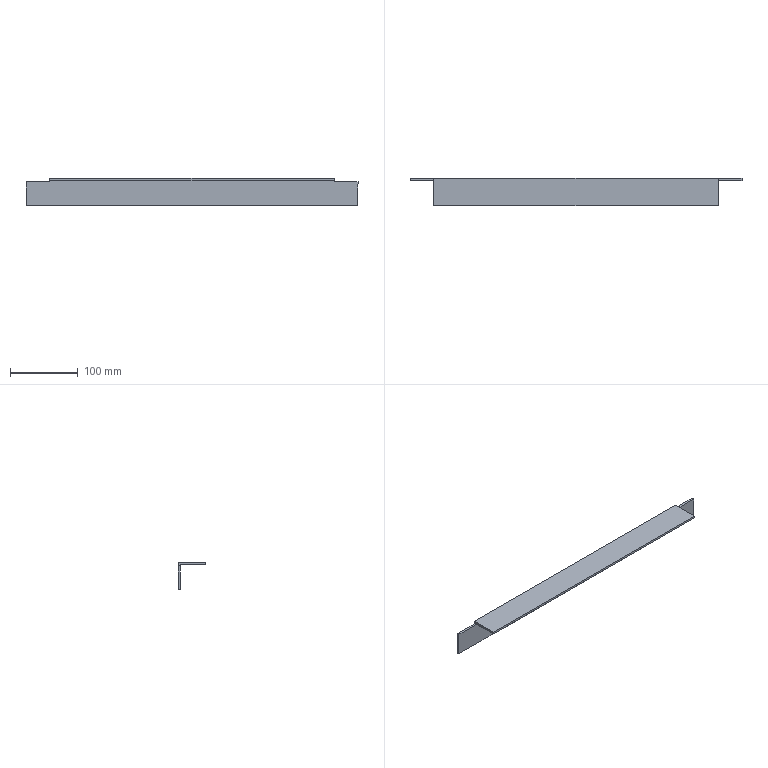Component | SolidWorks | LX-TSJ-13-1 | 1 solid | 12 faces | box 490 x 40 x 40 mm | volume 104370 mm3 | plane 12
STEP:
#1=COLOUR_RGB('',0.7922,0.8196,0.9333);
#2=FILL_AREA_STYLE_COLOUR('',#1);
#3=FILL_AREA_STYLE('',(#2));
#4=SURFACE_STYLE_FILL_AREA(#3);
#5=SURFACE_SIDE_STYLE('',(#4));
#6=SURFACE_STYLE_USAGE(.BOTH.,#5);
#7=PRESENTATION_STYLE_ASSIGNMENT((#6));
#8=CARTESIAN_POINT('',(2.637,-23.56,-6.468));
#9=VERTEX_POINT('',#8);
#10=CARTESIAN_POINT('',(-13.899,-23.56,-6.468));
#11=VERTEX_POINT('',#10);
#12=CARTESIAN_POINT('',(-15.276,-23.56,-6.468));
#13=DIRECTION('',(-1.,0.,0.));
#14=VECTOR('',#13,39.37);
#15=LINE('',#12,#14);
#16=EDGE_CURVE('',#9,#11,#15,.T.);
#17=ORIENTED_EDGE('',*,*,#16,.F.);
#18=CARTESIAN_POINT('',(2.637,-23.56,-6.665));
#19=VERTEX_POINT('',#18);
#20=CARTESIAN_POINT('',(2.637,-23.56,-8.043));
#21=DIRECTION('',(0.,0.,1.));
#22=VECTOR('',#21,39.37);
#23=LINE('',#20,#22);
#24=EDGE_CURVE('',#19,#9,#23,.T.);
#25=ORIENTED_EDGE('',*,*,#24,.F.);
#26=CARTESIAN_POINT('',(4.015,-23.56,-6.665));
#27=VERTEX_POINT('',#26);
#28=CARTESIAN_POINT('',(-15.276,-23.56,-6.665));
#29=DIRECTION('',(-1.,0.,0.));
#30=VECTOR('',#29,39.37);
#31=LINE('',#28,#30);
#32=EDGE_CURVE('',#27,#19,#31,.T.);
#33=ORIENTED_EDGE('',*,*,#32,.F.);
#34=CARTESIAN_POINT('',(4.015,-23.56,-8.043));
#35=VERTEX_POINT('',#34);
#36=CARTESIAN_POINT('',(4.015,-23.56,-8.043));
#37=DIRECTION('',(0.,0.,1.));
#38=VECTOR('',#37,39.37);
#39=LINE('',#36,#38);
#40=EDGE_CURVE('',#35,#27,#39,.T.);
#41=ORIENTED_EDGE('',*,*,#40,.F.);
#42=CARTESIAN_POINT('',(-15.276,-23.56,-8.043));
#43=VERTEX_POINT('',#42);
#44=CARTESIAN_POINT('',(-15.276,-23.56,-8.043));
#45=DIRECTION('',(1.,0.,-0.));
#46=VECTOR('',#45,39.37);
#47=LINE('',#44,#46);
#48=EDGE_CURVE('',#43,#35,#47,.T.);
#49=ORIENTED_EDGE('',*,*,#48,.F.);
#50=CARTESIAN_POINT('',(-15.276,-23.56,-6.665));
#51=VERTEX_POINT('',#50);
#52=CARTESIAN_POINT('',(-15.276,-23.56,-8.043));
#53=DIRECTION('',(-0.,0.,-1.));
#54=VECTOR('',#53,39.37);
#55=LINE('',#52,#54);
#56=EDGE_CURVE('',#51,#43,#55,.T.);
#57=ORIENTED_EDGE('',*,*,#56,.F.);
#58=CARTESIAN_POINT('',(-13.899,-23.56,-6.665));
#59=VERTEX_POINT('',#58);
#60=CARTESIAN_POINT('',(-15.276,-23.56,-6.665));
#61=DIRECTION('',(-1.,0.,0.));
#62=VECTOR('',#61,39.37);
#63=LINE('',#60,#62);
#64=EDGE_CURVE('',#59,#51,#63,.T.);
#65=ORIENTED_EDGE('',*,*,#64,.F.);
#66=CARTESIAN_POINT('',(-13.899,-23.56,-8.043));
#67=DIRECTION('',(-0.,0.,-1.));
#68=VECTOR('',#67,39.37);
#69=LINE('',#66,#68);
#70=EDGE_CURVE('',#11,#59,#69,.T.);
#71=ORIENTED_EDGE('',*,*,#70,.F.);
#72=EDGE_LOOP('',(#17,#25,#33,#41,#49,#57,#65,#71));
#73=FACE_OUTER_BOUND('',#72,.T.);
#74=CARTESIAN_POINT('',(-15.276,-23.56,-8.043));
#75=DIRECTION('',(0.,-1.,0.));
#76=DIRECTION('',(1.,0.,-0.));
#77=AXIS2_PLACEMENT_3D('',#74,#75,#76);
#78=PLANE('',#77);
#79=ADVANCED_FACE('',(#73),#78,.F.);
#80=ORIENTED_EDGE('',*,*,#16,.T.);
#81=CARTESIAN_POINT('',(-13.899,-25.134,-6.468));
#82=VERTEX_POINT('',#81);
#83=CARTESIAN_POINT('',(-13.899,-23.56,-6.468));
#84=DIRECTION('',(0.,1.,0.));
#85=VECTOR('',#84,39.37);
#86=LINE('',#83,#85);
#87=EDGE_CURVE('',#82,#11,#86,.T.);
#88=ORIENTED_EDGE('',*,*,#87,.F.);
#89=CARTESIAN_POINT('',(2.637,-25.134,-6.468));
#90=VERTEX_POINT('',#89);
#91=CARTESIAN_POINT('',(-15.276,-25.134,-6.468));
#92=DIRECTION('',(-1.,0.,0.));
#93=VECTOR('',#92,39.37);
#94=LINE('',#91,#93);
#95=EDGE_CURVE('',#90,#82,#94,.T.);
#96=ORIENTED_EDGE('',*,*,#95,.F.);
#97=CARTESIAN_POINT('',(2.637,-23.56,-6.468));
#98=DIRECTION('',(0.,-1.,0.));
#99=VECTOR('',#98,39.37);
#100=LINE('',#97,#99);
#101=EDGE_CURVE('',#9,#90,#100,.T.);
#102=ORIENTED_EDGE('',*,*,#101,.F.);
#103=EDGE_LOOP('',(#80,#88,#96,#102));
#104=FACE_OUTER_BOUND('',#103,.T.);
#105=CARTESIAN_POINT('',(-15.276,-23.56,-6.468));
#106=DIRECTION('',(-0.,0.,-1.));
#107=DIRECTION('',(-1.,0.,0.));
#108=AXIS2_PLACEMENT_3D('',#105,#106,#107);
#109=PLANE('',#108);
#110=ADVANCED_FACE('',(#104),#109,.F.);
#111=ORIENTED_EDGE('',*,*,#101,.T.);
#112=CARTESIAN_POINT('',(2.637,-25.134,-6.587));
#113=VERTEX_POINT('',#112);
#114=CARTESIAN_POINT('',(2.637,-25.134,-6.665));
#115=DIRECTION('',(0.,0.,1.));
#116=VECTOR('',#115,39.37);
#117=LINE('',#114,#116);
#118=EDGE_CURVE('',#113,#90,#117,.T.);
#119=ORIENTED_EDGE('',*,*,#118,.F.);
#120=CARTESIAN_POINT('',(2.637,-23.678,-6.587));
#121=VERTEX_POINT('',#120);
#122=CARTESIAN_POINT('',(2.637,-25.134,-6.587));
#123=DIRECTION('',(0.,-1.,0.));
#124=VECTOR('',#123,39.37);
#125=LINE('',#122,#124);
#126=EDGE_CURVE('',#121,#113,#125,.T.);
#127=ORIENTED_EDGE('',*,*,#126,.F.);
#128=CARTESIAN_POINT('',(2.637,-23.678,-6.665));
#129=VERTEX_POINT('',#128);
#130=CARTESIAN_POINT('',(2.637,-23.678,-6.665));
#131=DIRECTION('',(0.,0.,1.));
#132=VECTOR('',#131,39.37);
#133=LINE('',#130,#132);
#134=EDGE_CURVE('',#129,#121,#133,.T.);
#135=ORIENTED_EDGE('',*,*,#134,.F.);
#136=CARTESIAN_POINT('',(2.637,-25.134,-6.665));
#137=DIRECTION('',(0.,-1.,0.));
#138=VECTOR('',#137,39.37);
#139=LINE('',#136,#138);
#140=EDGE_CURVE('',#19,#129,#139,.T.);
#141=ORIENTED_EDGE('',*,*,#140,.F.);
#142=ORIENTED_EDGE('',*,*,#24,.T.);
#143=EDGE_LOOP('',(#111,#119,#127,#135,#141,#142));
#144=FACE_OUTER_BOUND('',#143,.T.);
#145=CARTESIAN_POINT('',(2.637,-25.134,-6.665));
#146=DIRECTION('',(-1.,0.,0.));
#147=DIRECTION('',(0.,0.,1.));
#148=AXIS2_PLACEMENT_3D('',#145,#146,#147);
#149=PLANE('',#148);
#150=ADVANCED_FACE('',(#144),#149,.F.);
#151=ORIENTED_EDGE('',*,*,#32,.T.);
#152=ORIENTED_EDGE('',*,*,#140,.T.);
#153=CARTESIAN_POINT('',(4.015,-23.678,-6.665));
#154=VERTEX_POINT('',#153);
#155=CARTESIAN_POINT('',(4.015,-23.678,-6.665));
#156=DIRECTION('',(1.,0.,-0.));
#157=VECTOR('',#156,39.37);
#158=LINE('',#155,#157);
#159=EDGE_CURVE('',#129,#154,#158,.T.);
#160=ORIENTED_EDGE('',*,*,#159,.T.);
#161=CARTESIAN_POINT('',(4.015,-23.56,-6.665));
#162=DIRECTION('',(0.,1.,0.));
#163=VECTOR('',#162,39.37);
#164=LINE('',#161,#163);
#165=EDGE_CURVE('',#154,#27,#164,.T.);
#166=ORIENTED_EDGE('',*,*,#165,.T.);
#167=EDGE_LOOP('',(#151,#152,#160,#166));
#168=FACE_OUTER_BOUND('',#167,.T.);
#169=CARTESIAN_POINT('',(4.015,-23.56,-6.665));
#170=DIRECTION('',(0.,0.,1.));
#171=DIRECTION('',(1.,0.,-0.));
#172=AXIS2_PLACEMENT_3D('',#169,#170,#171);
#173=PLANE('',#172);
#174=ADVANCED_FACE('',(#168),#173,.T.);
#175=CARTESIAN_POINT('',(4.015,-23.678,-8.043));
#176=VERTEX_POINT('',#175);
#177=CARTESIAN_POINT('',(4.015,-23.678,-8.043));
#178=DIRECTION('',(0.,0.,1.));
#179=VECTOR('',#178,39.37);
#180=LINE('',#177,#179);
#181=EDGE_CURVE('',#176,#154,#180,.T.);
#182=ORIENTED_EDGE('',*,*,#181,.F.);
#183=CARTESIAN_POINT('',(4.015,-23.56,-8.043));
#184=DIRECTION('',(0.,-1.,0.));
#185=VECTOR('',#184,39.37);
#186=LINE('',#183,#185);
#187=EDGE_CURVE('',#35,#176,#186,.T.);
#188=ORIENTED_EDGE('',*,*,#187,.F.);
#189=ORIENTED_EDGE('',*,*,#40,.T.);
#190=ORIENTED_EDGE('',*,*,#165,.F.);
#191=EDGE_LOOP('',(#182,#188,#189,#190));
#192=FACE_OUTER_BOUND('',#191,.T.);
#193=CARTESIAN_POINT('',(4.015,-23.56,-8.043));
#194=DIRECTION('',(-1.,0.,0.));
#195=DIRECTION('',(0.,0.,1.));
#196=AXIS2_PLACEMENT_3D('',#193,#194,#195);
#197=PLANE('',#196);
#198=ADVANCED_FACE('',(#192),#197,.F.);
#199=CARTESIAN_POINT('',(-15.276,-23.678,-8.043));
#200=VERTEX_POINT('',#199);
#201=CARTESIAN_POINT('',(-15.276,-23.678,-8.043));
#202=DIRECTION('',(1.,0.,-0.));
#203=VECTOR('',#202,39.37);
#204=LINE('',#201,#203);
#205=EDGE_CURVE('',#200,#176,#204,.T.);
#206=ORIENTED_EDGE('',*,*,#205,.F.);
#207=CARTESIAN_POINT('',(-15.276,-23.56,-8.043));
#208=DIRECTION('',(0.,-1.,0.));
#209=VECTOR('',#208,39.37);
#210=LINE('',#207,#209);
#211=EDGE_CURVE('',#43,#200,#210,.T.);
#212=ORIENTED_EDGE('',*,*,#211,.F.);
#213=ORIENTED_EDGE('',*,*,#48,.T.);
#214=ORIENTED_EDGE('',*,*,#187,.T.);
#215=EDGE_LOOP('',(#206,#212,#213,#214));
#216=FACE_OUTER_BOUND('',#215,.T.);
#217=CARTESIAN_POINT('',(-15.276,-23.56,-8.043));
#218=DIRECTION('',(0.,0.,1.));
#219=DIRECTION('',(1.,0.,-0.));
#220=AXIS2_PLACEMENT_3D('',#217,#218,#219);
#221=PLANE('',#220);
#222=ADVANCED_FACE('',(#216),#221,.F.);
#223=ORIENTED_EDGE('',*,*,#211,.T.);
#224=CARTESIAN_POINT('',(-15.276,-23.678,-6.665));
#225=VERTEX_POINT('',#224);
#226=CARTESIAN_POINT('',(-15.276,-23.678,-8.043));
#227=DIRECTION('',(0.,0.,1.));
#228=VECTOR('',#227,39.37);
#229=LINE('',#226,#228);
#230=EDGE_CURVE('',#200,#225,#229,.T.);
#231=ORIENTED_EDGE('',*,*,#230,.T.);
#232=CARTESIAN_POINT('',(-15.276,-23.56,-6.665));
#233=DIRECTION('',(0.,1.,0.));
#234=VECTOR('',#233,39.37);
#235=LINE('',#232,#234);
#236=EDGE_CURVE('',#225,#51,#235,.T.);
#237=ORIENTED_EDGE('',*,*,#236,.T.);
#238=ORIENTED_EDGE('',*,*,#56,.T.);
#239=EDGE_LOOP('',(#223,#231,#237,#238));
#240=FACE_OUTER_BOUND('',#239,.T.);
#241=CARTESIAN_POINT('',(-15.276,-23.56,-8.043));
#242=DIRECTION('',(-1.,0.,0.));
#243=DIRECTION('',(0.,0.,1.));
#244=AXIS2_PLACEMENT_3D('',#241,#242,#243);
#245=PLANE('',#244);
#246=ADVANCED_FACE('',(#240),#245,.T.);
#247=ORIENTED_EDGE('',*,*,#64,.T.);
#248=ORIENTED_EDGE('',*,*,#236,.F.);
#249=CARTESIAN_POINT('',(-13.899,-23.678,-6.665));
#250=VERTEX_POINT('',#249);
#251=CARTESIAN_POINT('',(4.015,-23.678,-6.665));
#252=DIRECTION('',(-1.,0.,0.));
#253=VECTOR('',#252,39.37);
#254=LINE('',#251,#253);
#255=EDGE_CURVE('',#250,#225,#254,.T.);
#256=ORIENTED_EDGE('',*,*,#255,.F.);
#257=CARTESIAN_POINT('',(-13.899,-23.56,-6.665));
#258=DIRECTION('',(0.,-1.,0.));
#259=VECTOR('',#258,39.37);
#260=LINE('',#257,#259);
#261=EDGE_CURVE('',#59,#250,#260,.T.);
#262=ORIENTED_EDGE('',*,*,#261,.F.);
#263=EDGE_LOOP('',(#247,#248,#256,#262));
#264=FACE_OUTER_BOUND('',#263,.T.);
#265=CARTESIAN_POINT('',(4.015,-23.56,-6.665));
#266=DIRECTION('',(-0.,0.,-1.));
#267=DIRECTION('',(-1.,0.,0.));
#268=AXIS2_PLACEMENT_3D('',#265,#266,#267);
#269=PLANE('',#268);
#270=ADVANCED_FACE('',(#264),#269,.F.);
#271=CARTESIAN_POINT('',(-13.899,-23.678,-6.587));
#272=VERTEX_POINT('',#271);
#273=CARTESIAN_POINT('',(-13.899,-23.678,-6.665));
#274=DIRECTION('',(-0.,0.,-1.));
#275=VECTOR('',#274,39.37);
#276=LINE('',#273,#275);
#277=EDGE_CURVE('',#272,#250,#276,.T.);
#278=ORIENTED_EDGE('',*,*,#277,.F.);
#279=CARTESIAN_POINT('',(-13.899,-25.134,-6.587));
#280=VERTEX_POINT('',#279);
#281=CARTESIAN_POINT('',(-13.899,-25.134,-6.587));
#282=DIRECTION('',(0.,1.,0.));
#283=VECTOR('',#282,39.37);
#284=LINE('',#281,#283);
#285=EDGE_CURVE('',#280,#272,#284,.T.);
#286=ORIENTED_EDGE('',*,*,#285,.F.);
#287=CARTESIAN_POINT('',(-13.899,-25.134,-6.665));
#288=DIRECTION('',(-0.,0.,-1.));
#289=VECTOR('',#288,39.37);
#290=LINE('',#287,#289);
#291=EDGE_CURVE('',#82,#280,#290,.T.);
#292=ORIENTED_EDGE('',*,*,#291,.F.);
#293=ORIENTED_EDGE('',*,*,#87,.T.);
#294=ORIENTED_EDGE('',*,*,#70,.T.);
#295=ORIENTED_EDGE('',*,*,#261,.T.);
#296=EDGE_LOOP('',(#278,#286,#292,#293,#294,#295));
#297=FACE_OUTER_BOUND('',#296,.T.);
#298=CARTESIAN_POINT('',(-13.899,-25.134,-6.665));
#299=DIRECTION('',(1.,0.,-0.));
#300=DIRECTION('',(-0.,0.,-1.));
#301=AXIS2_PLACEMENT_3D('',#298,#299,#300);
#302=PLANE('',#301);
#303=ADVANCED_FACE('',(#297),#302,.F.);
#304=ORIENTED_EDGE('',*,*,#118,.T.);
#305=ORIENTED_EDGE('',*,*,#95,.T.);
#306=ORIENTED_EDGE('',*,*,#291,.T.);
#307=CARTESIAN_POINT('',(-15.276,-25.134,-6.587));
#308=DIRECTION('',(-1.,0.,0.));
#309=VECTOR('',#308,39.37);
#310=LINE('',#307,#309);
#311=EDGE_CURVE('',#113,#280,#310,.T.);
#312=ORIENTED_EDGE('',*,*,#311,.F.);
#313=EDGE_LOOP('',(#304,#305,#306,#312));
#314=FACE_OUTER_BOUND('',#313,.T.);
#315=CARTESIAN_POINT('',(-15.276,-25.134,-6.587));
#316=DIRECTION('',(0.,1.,0.));
#317=DIRECTION('',(-1.,0.,0.));
#318=AXIS2_PLACEMENT_3D('',#315,#316,#317);
#319=PLANE('',#318);
#320=ADVANCED_FACE('',(#314),#319,.F.);
#321=ORIENTED_EDGE('',*,*,#126,.T.);
#322=ORIENTED_EDGE('',*,*,#311,.T.);
#323=ORIENTED_EDGE('',*,*,#285,.T.);
#324=CARTESIAN_POINT('',(-15.276,-23.678,-6.587));
#325=DIRECTION('',(-1.,0.,0.));
#326=VECTOR('',#325,39.37);
#327=LINE('',#324,#326);
#328=EDGE_CURVE('',#121,#272,#327,.T.);
#329=ORIENTED_EDGE('',*,*,#328,.F.);
#330=EDGE_LOOP('',(#321,#322,#323,#329));
#331=FACE_OUTER_BOUND('',#330,.T.);
#332=CARTESIAN_POINT('',(-15.276,-23.678,-6.587));
#333=DIRECTION('',(0.,0.,1.));
#334=DIRECTION('',(1.,0.,-0.));
#335=AXIS2_PLACEMENT_3D('',#332,#333,#334);
#336=PLANE('',#335);
#337=ADVANCED_FACE('',(#331),#336,.F.);
#338=ORIENTED_EDGE('',*,*,#134,.T.);
#339=ORIENTED_EDGE('',*,*,#328,.T.);
#340=ORIENTED_EDGE('',*,*,#277,.T.);
#341=ORIENTED_EDGE('',*,*,#255,.T.);
#342=ORIENTED_EDGE('',*,*,#230,.F.);
#343=ORIENTED_EDGE('',*,*,#205,.T.);
#344=ORIENTED_EDGE('',*,*,#181,.T.);
#345=ORIENTED_EDGE('',*,*,#159,.F.);
#346=EDGE_LOOP('',(#338,#339,#340,#341,#342,#343,#344,#345));
#347=FACE_OUTER_BOUND('',#346,.T.);
#348=CARTESIAN_POINT('',(-15.276,-23.678,-8.043));
#349=DIRECTION('',(0.,1.,0.));
#350=DIRECTION('',(-1.,0.,0.));
#351=AXIS2_PLACEMENT_3D('',#348,#349,#350);
#352=PLANE('',#351);
#353=ADVANCED_FACE('',(#347),#352,.F.);
#354=CLOSED_SHELL('',(#79,#110,#150,#174,#198,#222,#246,#270,#303,#320,#337,#353));
#355=MANIFOLD_SOLID_BREP('',#354);
#356=STYLED_ITEM('',(#7),#355);
#357=(LENGTH_UNIT()NAMED_UNIT(*)SI_UNIT($,.METRE.));
#358=LENGTH_MEASURE_WITH_UNIT(LENGTH_MEASURE(0.0254),#357);
#359=DIMENSIONAL_EXPONENTS(1.,0.,0.,0.,0.,0.,0.);
#360=(CONVERSION_BASED_UNIT('',#358)LENGTH_UNIT()NAMED_UNIT(#359));
#361=UNCERTAINTY_MEASURE_WITH_UNIT(LENGTH_MEASURE(0.00001),#360,'','');
#362=(NAMED_UNIT(*)PLANE_ANGLE_UNIT()SI_UNIT($,.RADIAN.));
#363=(NAMED_UNIT(*)SI_UNIT($,.STERADIAN.)SOLID_ANGLE_UNIT());
#364=(GEOMETRIC_REPRESENTATION_CONTEXT(3)GLOBAL_UNCERTAINTY_ASSIGNED_CONTEXT((#361))GLOBAL_UNIT_ASSIGNED_CONTEXT((#360,#362,#363))REPRESENTATION_CONTEXT('',''));
#365=MECHANICAL_DESIGN_GEOMETRIC_PRESENTATION_REPRESENTATION('',(#356),#364);
#366=PRESENTATION_LAYER_ASSIGNMENT('','',(#356));
#367=CARTESIAN_POINT('',(0.,0.,0.));
#368=DIRECTION('',(0.,0.,1.));
#369=DIRECTION('',(1.,0.,0.));
#370=AXIS2_PLACEMENT_3D('',#367,#368,#369);
#371=(LENGTH_UNIT()NAMED_UNIT(*)SI_UNIT($,.METRE.));
#372=LENGTH_MEASURE_WITH_UNIT(LENGTH_MEASURE(0.0254),#371);
#373=DIMENSIONAL_EXPONENTS(1.,0.,0.,0.,0.,0.,0.);
#374=(CONVERSION_BASED_UNIT('',#372)LENGTH_UNIT()NAMED_UNIT(#373));
#375=UNCERTAINTY_MEASURE_WITH_UNIT(LENGTH_MEASURE(0.00001),#374,'','');
#376=(NAMED_UNIT(*)PLANE_ANGLE_UNIT()SI_UNIT($,.RADIAN.));
#377=(NAMED_UNIT(*)SI_UNIT($,.STERADIAN.)SOLID_ANGLE_UNIT());
#378=(GEOMETRIC_REPRESENTATION_CONTEXT(3)GLOBAL_UNCERTAINTY_ASSIGNED_CONTEXT((#375))GLOBAL_UNIT_ASSIGNED_CONTEXT((#374,#376,#377))REPRESENTATION_CONTEXT('',''));
#379=ADVANCED_BREP_SHAPE_REPRESENTATION('',(#355,#370),#378);